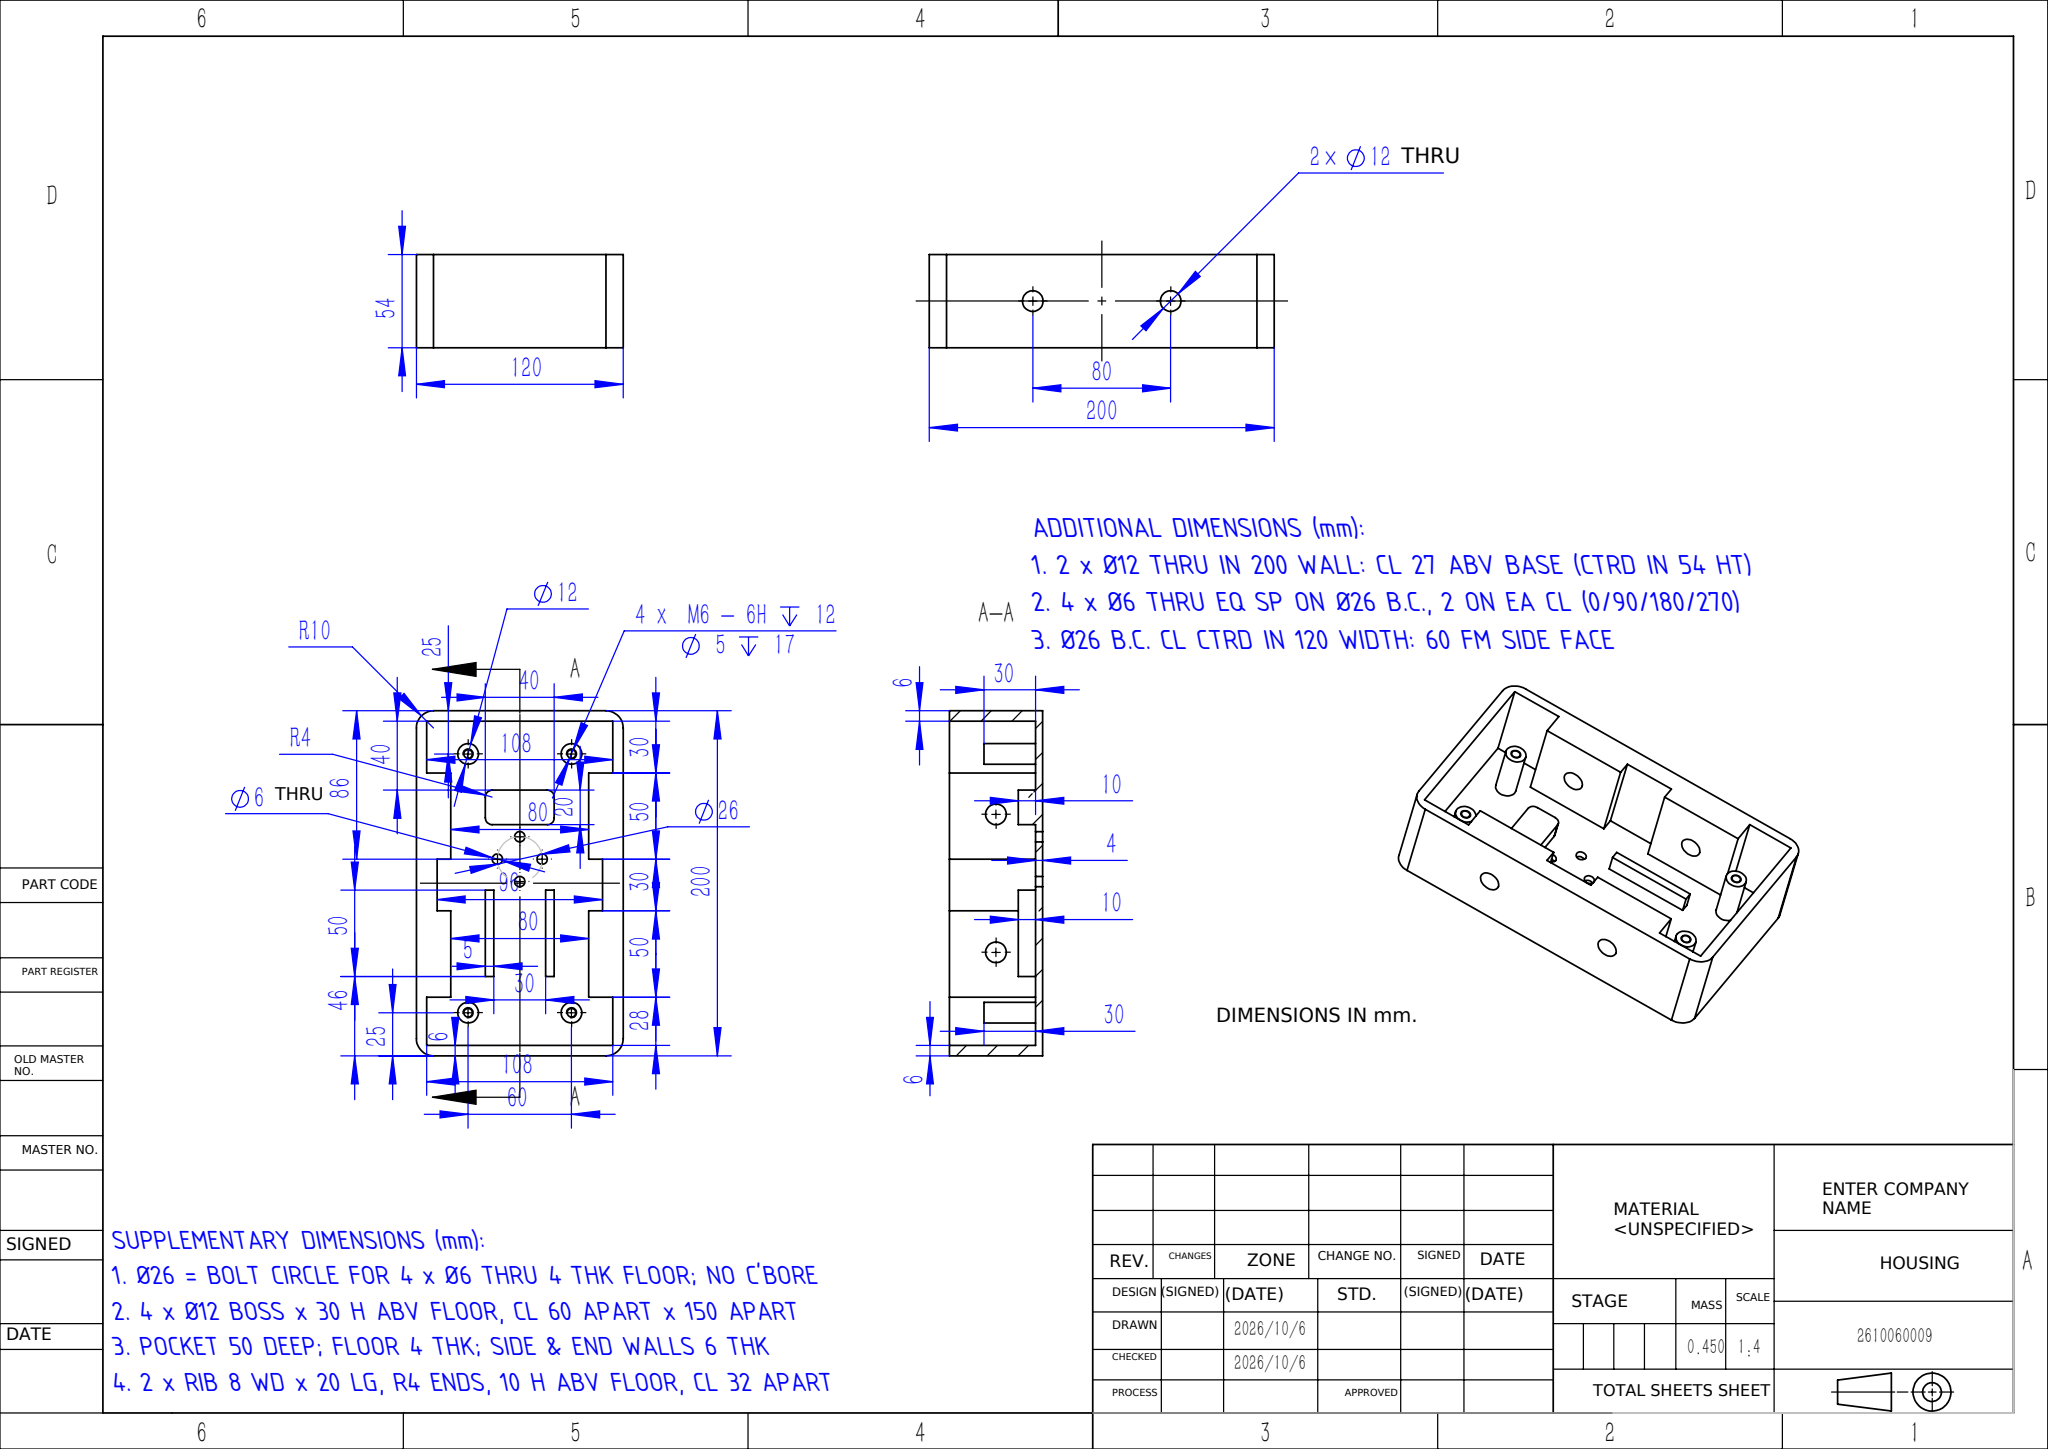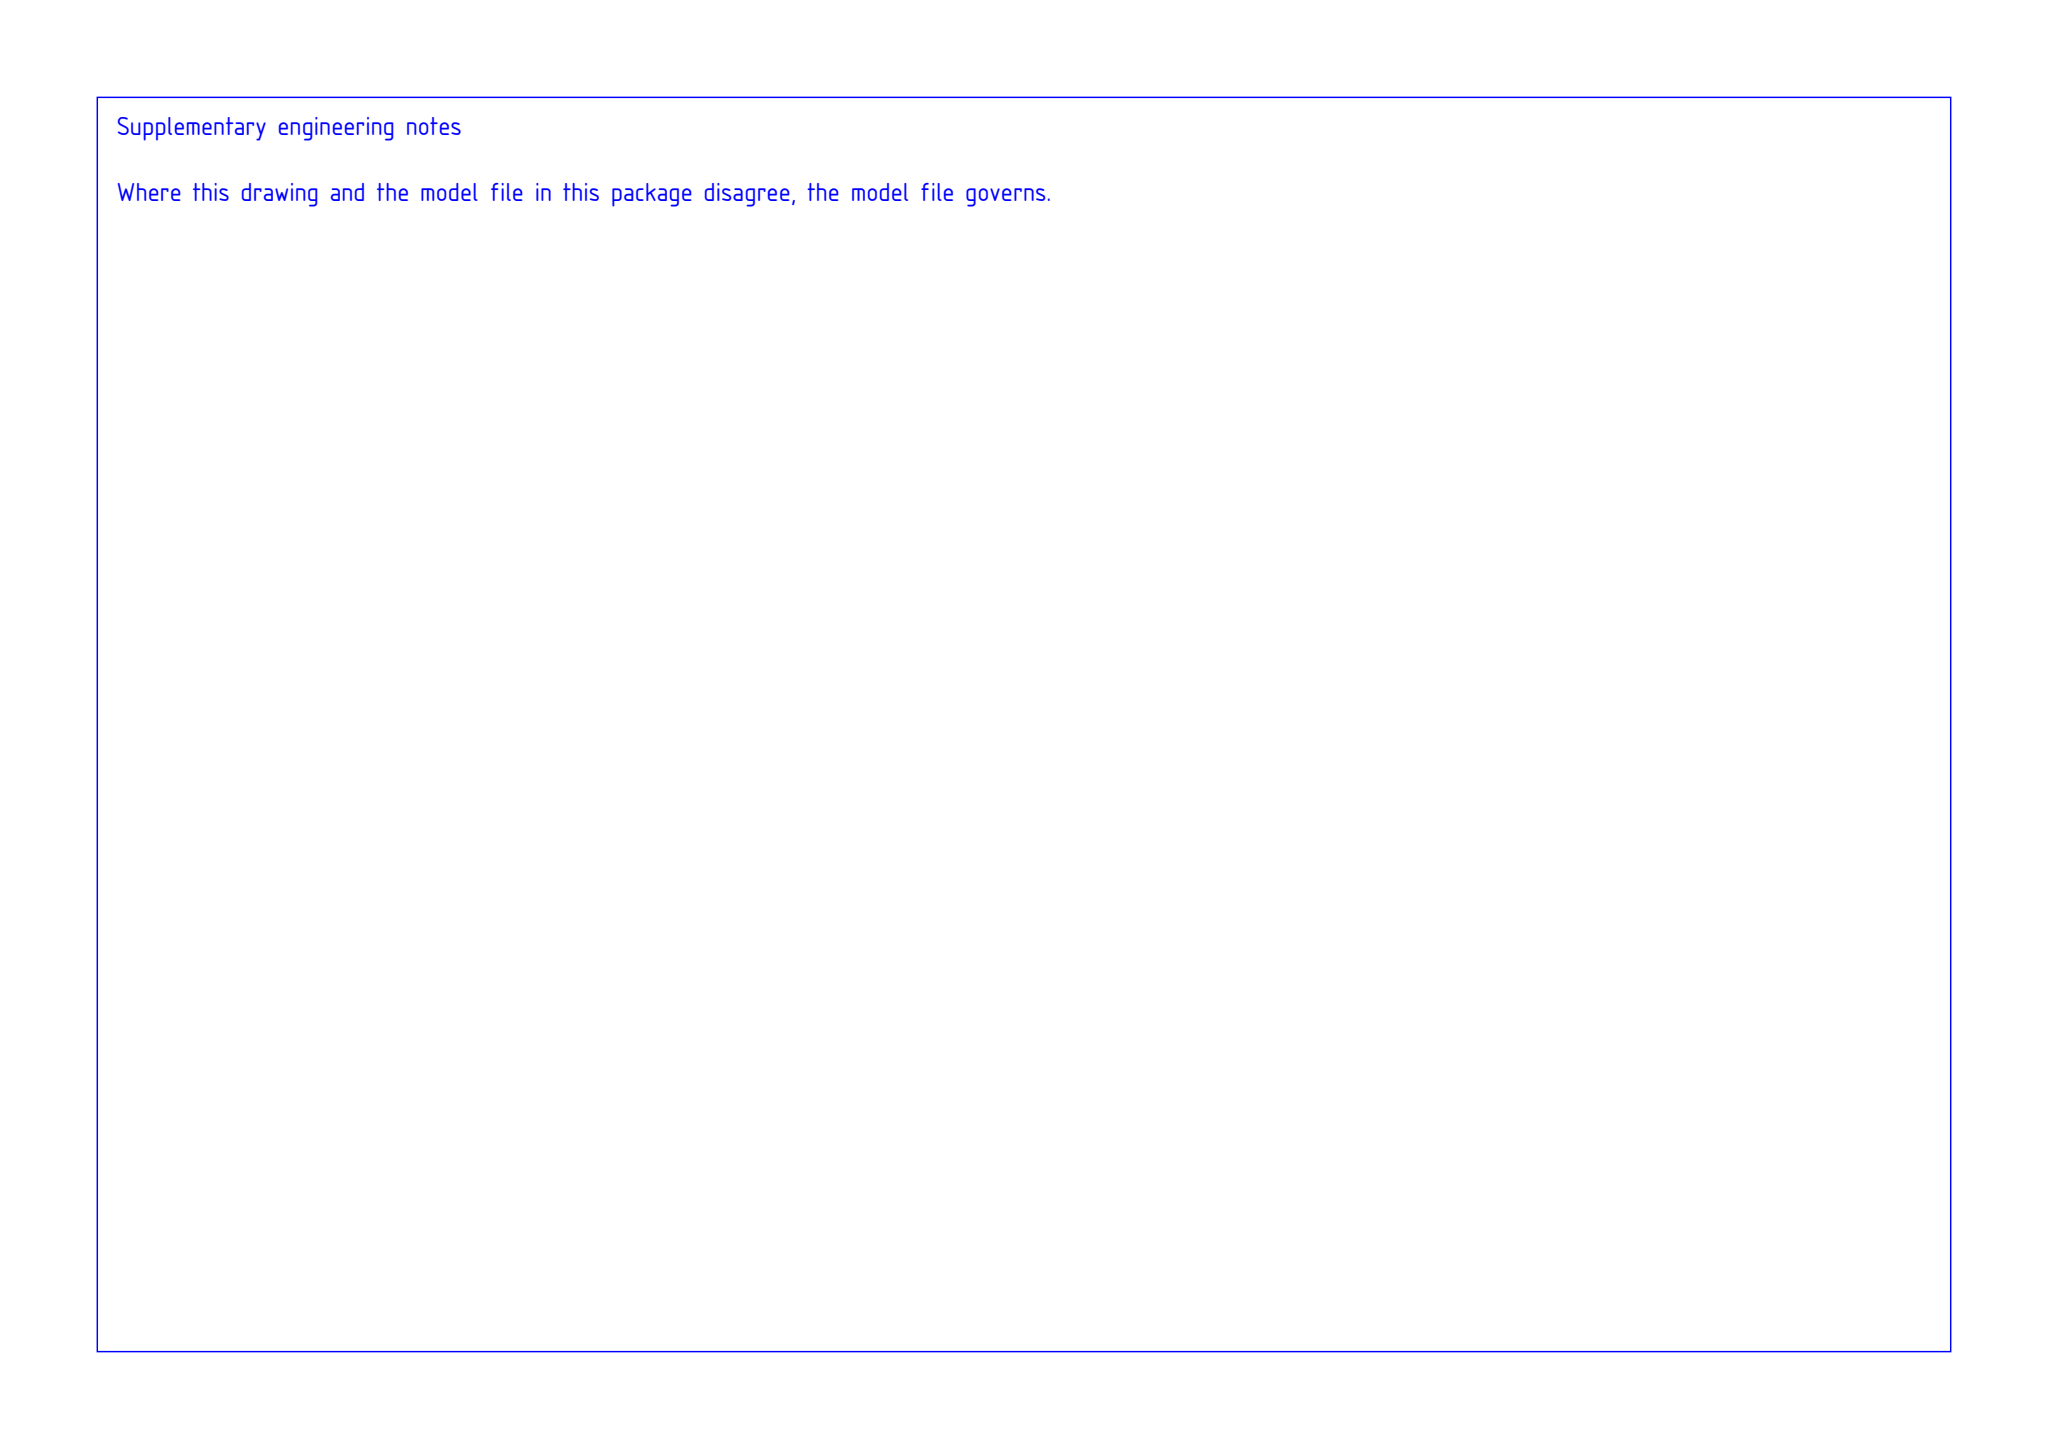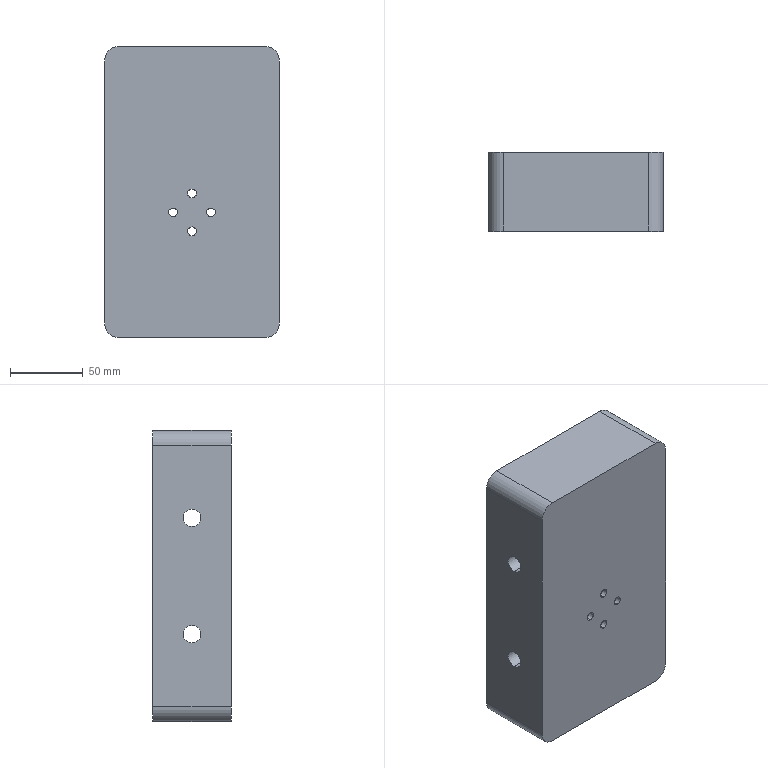Part | SolidWorks | mm | 1 solid | 94 faces | box 120 x 54 x 200 mm | volume 449724 mm3 | plane 46 | cylinder 40 | cone 8 | commonest cylinder face diameters 12 x16 6 x8 5 x8 20 x4 8 x4
build123d program:
from build123d import *

# Parameters (mm, degrees)
BOSS_EXTRUDE1_DEPTH   = 50
BOSS_EXTRUDE2_START   = 4
BOSS_EXTRUDE2_DEPTH   = 4
SKETCH3_R             = 6
BOSS_EXTRUDE3_DEPTH   = 30
M6_TAPPED_HOLE1_D     = 5
M6_TAPPED_HOLE1_DEPTH = 17
M6_TAPPED_HOLE1_TIP   = 1.502
SKETCH8_W             = 40
SKETCH8_H             = 20
BOSS_EXTRUDE4_DEPTH   = 10
FILLET1_R             = 4
SKETCH9_W             = 5
SKETCH9_H             = 50
BOSS_EXTRUDE5_DEPTH   = 10
SKETCH10_R            = 6
CUT_EXTRUDE1_DEPTH    = 165.012
SKETCH11_R            = 3
CUT_EXTRUDE2_DEPTH    = 127.886


with BuildPart() as part:
    # Sketch1 → Boss-Extrude1 (new body)
    with BuildSketch(Plane(origin=(0, 0, 0), x_dir=(1, 0, 0), z_dir=(0, 1, 0))):
        with BuildLine():
            Line((-50, -100), (50, -100))
            ThreePointArc((50, -100), (57.071, -97.071), (60, -90))
            Line((60, -90), (60, 90))
            ThreePointArc((60, 90), (57.071, 97.071), (50, 100))
            Line((50, 100), (-50, 100))
            ThreePointArc((-50, 100), (-57.071, 97.071), (-60, 90))
            Line((-60, 90), (-60, -90))
            ThreePointArc((-60, -90), (-57.071, -97.071), (-50, -100))
        make_face()
        Polygon((-54, 94), (54, 94), (54, 64), (40, 64), (40, 14), (48, 14), (48, -16), (40, -16), (40, -66), (54, -66), (54, -94), (-54, -94), (-54, -66), (-40, -66), (-40, -16), (-48, -16), (-48, 14), (-40, 14), (-40, 64), (-54, 64), align=None, mode=Mode.SUBTRACT)
    extrude(amount=BOSS_EXTRUDE1_DEPTH)

    # Sketch2 → Boss-Extrude2 (add)
    with BuildSketch(Plane.XZ.offset(BOSS_EXTRUDE2_START)):
        with BuildLine():
            Line((60, 90), (60, -90))
            ThreePointArc((60, -90), (57.071, -97.071), (50, -100))
            Line((50, -100), (-50, -100))
            ThreePointArc((-50, -100), (-57.071, -97.071), (-60, -90))
            Line((-60, -90), (-60, 90))
            ThreePointArc((-60, 90), (-57.071, 97.071), (-50, 100))
            Line((-50, 100), (50, 100))
            ThreePointArc((50, 100), (57.071, 97.071), (60, 90))
        make_face()
    extrude(amount=-BOSS_EXTRUDE2_DEPTH)

    # Sketch3 → Boss-Extrude3 (add)
    with BuildSketch(Plane(origin=(0, 0, 0), x_dir=(1, 0, 0), z_dir=(0, 1, 0))):
        with Locations(Location((-30, 75, 0), (0, 0, 90))):
            Circle(SKETCH3_R)
        with Locations(Location((30, 75, 0), (0, 0, 90))):
            Circle(SKETCH3_R)
        with Locations(Location((30, -75, 0), (0, 0, 90))):
            Circle(SKETCH3_R)
        with Locations(Location((-30, -75, 0), (0, 0, 90))):
            Circle(SKETCH3_R)
    extrude(amount=BOSS_EXTRUDE3_DEPTH)

    # M6 Tapped Hole1
    with Locations(Plane(origin=(0, 30, 0), x_dir=(1, 0, 0), z_dir=(0, 1, 0))):
        with Locations((-30, 75), (30, 75), (-30, -75), (30, -75)):
            Hole(M6_TAPPED_HOLE1_D / 2, depth=M6_TAPPED_HOLE1_DEPTH)
            with Locations((0, 0, -(M6_TAPPED_HOLE1_DEPTH + M6_TAPPED_HOLE1_TIP / 2))):  # 118° drill point
                Cone(0, M6_TAPPED_HOLE1_D / 2, M6_TAPPED_HOLE1_TIP, mode=Mode.SUBTRACT)

    # Sketch8 → Boss-Extrude4 (add)
    with BuildSketch(Plane(origin=(0, 0, 0), x_dir=(1, 0, 0), z_dir=(0, 1, 0))):
        with Locations((0, 44)):
            Rectangle(SKETCH8_W, SKETCH8_H)
    extrude(amount=BOSS_EXTRUDE4_DEPTH)

    # Fillet1
    fillet1_edges = [part.edges().sort_by_distance(p)[0] for p in [
        (-20, 5, -54),
        (-20, 5, -34),
        (20, 5, -34),
        (20, 5, -54),
    ]]
    fillet(fillet1_edges, radius=FILLET1_R)

    # Sketch9 → Boss-Extrude5 (add)
    with BuildSketch(Plane(origin=(0, 0, 0), x_dir=(1, 0, 0), z_dir=(0, 1, 0))):
        with Locations((-17.5, -29)):
            Rectangle(SKETCH9_W, SKETCH9_H)
        with Locations((17.5, -29)):
            Rectangle(SKETCH9_W, SKETCH9_H)
    extrude(amount=BOSS_EXTRUDE5_DEPTH)

    # Sketch10 → Cut-Extrude1 (cut, through all)
    with BuildSketch(Plane.ZY.offset(60)):
        with Locations((-40, 23)):
            Circle(SKETCH10_R)
        with Locations((40, 23)):
            Circle(SKETCH10_R)
    extrude(amount=-CUT_EXTRUDE1_DEPTH, mode=Mode.SUBTRACT)

    # Sketch11 → Cut-Extrude2 (cut, through all)
    with BuildSketch(Plane(origin=(0, 0, 0), x_dir=(1, 0, 0), z_dir=(0, 1, 0))):
        with Locations(Location((0, 27, 0), (0, 0, 270))):
            Circle(SKETCH11_R)
        with Locations(Location((13, 14, 0), (0, 0, 270))):
            Circle(SKETCH11_R)
        with Locations(Location((0, 1, 0), (0, 0, 270))):
            Circle(SKETCH11_R)
        with Locations(Location((-13, 14, 0), (0, 0, 270))):
            Circle(SKETCH11_R)
    extrude(amount=-CUT_EXTRUDE2_DEPTH, mode=Mode.SUBTRACT)


solid = part.part